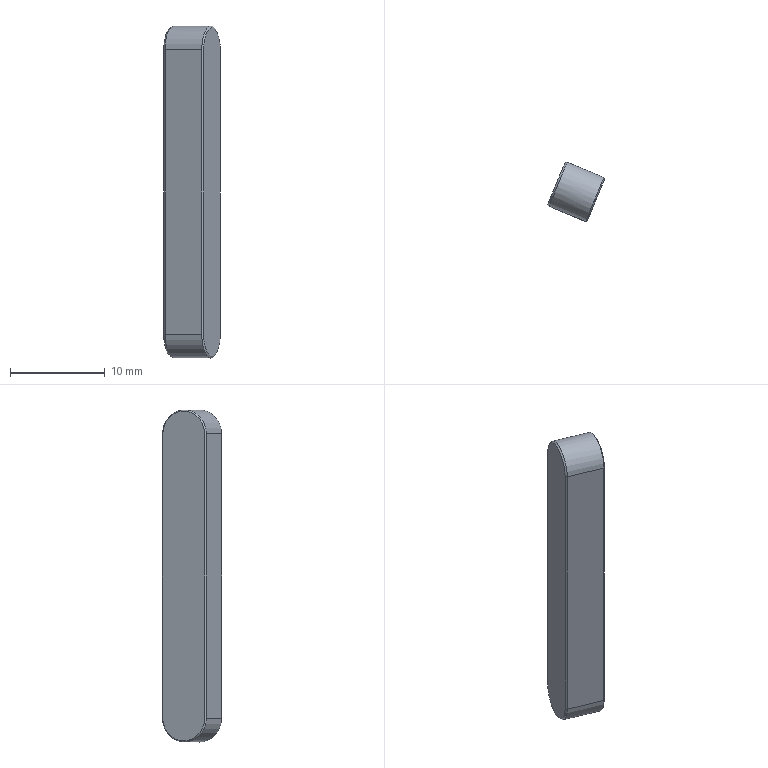Component | SolidWorks | 170423A4-ConveyorSynchronousPulleyAssembly-1_170423A4-Key5x30-1 | 1 solid | 17 faces | box 5.95 x 6.22 x 35 mm | volume 762 mm3 | plane 8 | cone 6 | cylinder 3 | commonest cylinder face diameters 5 x3
build123d program:
from build123d import *
from OCP.BRepFilletAPI import BRepFilletAPI_MakeChamfer

# Parameters (mm, degrees)
BOSS_EXTRUDE1_DEPTH = 4.5
CHAMFER1_SIZE       = 0.2
CHAMFER1_SIZE2      = 0.1155


with BuildPart() as part:
    # Sketch1 → Boss-Extrude1 (new body)
    with BuildSketch(Plane.XY):
        with BuildLine():
            Line((-15, 2.5), (15, 2.5))
            ThreePointArc((15, 2.5), (17.5, 0), (15, -2.5))
            Line((15, -2.5), (-15, -2.5))
            ThreePointArc((-15, -2.5), (-17.5, 0), (-15, 2.5))
        make_face()
    extrude(amount=BOSS_EXTRUDE1_DEPTH)

    # Chamfer1: one chamfer whose edges measure the first distance from different faces: ONE call of the kernel's chamfer builder (chamfer() names one face for all edges)
    chamfer1_edges_1 = [part.edges().sort_by_distance(p)[0] for p in [
        (17.5, 0, 4.5),
    ]]
    chamfer1_side_1 = [part.faces().sort_by_distance(p)[0] for p in [
        (17.5, 0, 2.25),
    ]]
    chamfer1_edges_2 = [part.edges().sort_by_distance(p)[0] for p in [
        (0, 2.5, 4.5),
    ]]
    chamfer1_side_2 = [part.faces().sort_by_distance(p)[0] for p in [
        (0, 2.5, 2.25),
    ]]
    chamfer1_edges_3 = [part.edges().sort_by_distance(p)[0] for p in [
        (-17.5, 0, 4.5),
    ]]
    chamfer1_side_3 = [part.faces().sort_by_distance(p)[0] for p in [
        (-17.5, 0, 2.25),
    ]]
    chamfer1_edges_4 = [part.edges().sort_by_distance(p)[0] for p in [
        (0, 2.5, 0),
        (17.5, 0, 0),
        (0, -2.5, 0),
        (-17.5, 0, 0),
    ]]
    chamfer1_side_4 = [part.faces().sort_by_distance(p)[0] for p in [
        (0, 0, 0),
    ]]
    chamfer1_edges_5 = [part.edges().sort_by_distance(p)[0] for p in [
        (0, -2.5, 4.5),
    ]]
    chamfer1_side_5 = [part.faces().sort_by_distance(p)[0] for p in [
        (0, -2.5, 2.25),
    ]]
    chamfer1 = BRepFilletAPI_MakeChamfer(part.part.solid().wrapped)
    for e in chamfer1_edges_1:
        chamfer1.Add(CHAMFER1_SIZE, CHAMFER1_SIZE2, e.wrapped, chamfer1_side_1[0].wrapped)  # the first distance lies on this face
    for e in chamfer1_edges_2:
        chamfer1.Add(CHAMFER1_SIZE, CHAMFER1_SIZE2, e.wrapped, chamfer1_side_2[0].wrapped)  # the first distance lies on this face
    for e in chamfer1_edges_3:
        chamfer1.Add(CHAMFER1_SIZE, CHAMFER1_SIZE2, e.wrapped, chamfer1_side_3[0].wrapped)  # the first distance lies on this face
    for e in chamfer1_edges_4:
        chamfer1.Add(CHAMFER1_SIZE, CHAMFER1_SIZE2, e.wrapped, chamfer1_side_4[0].wrapped)  # the first distance lies on this face
    for e in chamfer1_edges_5:
        chamfer1.Add(CHAMFER1_SIZE, CHAMFER1_SIZE2, e.wrapped, chamfer1_side_5[0].wrapped)  # the first distance lies on this face
    add(Compound.cast(chamfer1.Shape()), mode=Mode.REPLACE)


solid = part.part

# Placed as in the assembly
solid = solid.moved(Location((108.067, -124.236, 444), (-90, -67.477, -90)))
STEP:
#1=COLOUR_RGB('',0.7922,0.8196,0.9333);
#2=FILL_AREA_STYLE_COLOUR('',#1);
#3=FILL_AREA_STYLE('',(#2));
#4=SURFACE_STYLE_FILL_AREA(#3);
#5=SURFACE_SIDE_STYLE('',(#4));
#6=SURFACE_STYLE_USAGE(.BOTH.,#5);
#7=PRESENTATION_STYLE_ASSIGNMENT((#6));
#8=CARTESIAN_POINT('',(4.091,-4.823,16.796));
#9=VERTEX_POINT('',#8);
#10=CARTESIAN_POINT('',(4.055,-4.91,16.89));
#11=VERTEX_POINT('',#10);
#12=CARTESIAN_POINT('',(4.091,-4.823,16.89));
#13=DIRECTION('',(-0.9237,0.383,0.));
#14=DIRECTION('',(0.,-0.,1.));
#15=AXIS2_PLACEMENT_3D('',#12,#13,#14);
#16=CIRCLE('',#15,0.09388);
#17=EDGE_CURVE('',#9,#11,#16,.T.);
#18=ORIENTED_EDGE('',*,*,#17,.F.);
#19=CARTESIAN_POINT('',(4.098,-4.826,16.791));
#20=VERTEX_POINT('',#19);
#21=CARTESIAN_POINT('',(4.091,-4.823,16.796));
#22=DIRECTION('',(0.8,-0.3317,-0.5));
#23=VECTOR('',#22,39.37);
#24=LINE('',#21,#23);
#25=EDGE_CURVE('',#9,#20,#24,.T.);
#26=ORIENTED_EDGE('',*,*,#25,.T.);
#27=CARTESIAN_POINT('',(4.061,-4.917,16.89));
#28=VERTEX_POINT('',#27);
#29=CARTESIAN_POINT('',(4.098,-4.826,16.89));
#30=DIRECTION('',(0.9237,-0.383,-0.));
#31=DIRECTION('',(0.,-0.,1.));
#32=AXIS2_PLACEMENT_3D('',#29,#30,#31);
#33=CIRCLE('',#32,0.09843);
#34=EDGE_CURVE('',#28,#20,#33,.T.);
#35=ORIENTED_EDGE('',*,*,#34,.F.);
#36=CARTESIAN_POINT('',(4.061,-4.917,16.89));
#37=DIRECTION('',(-0.6084,0.7936,0.));
#38=VECTOR('',#37,39.37);
#39=LINE('',#36,#38);
#40=EDGE_CURVE('',#28,#11,#39,.T.);
#41=ORIENTED_EDGE('',*,*,#40,.T.);
#42=EDGE_LOOP('',(#18,#26,#35,#41));
#43=FACE_OUTER_BOUND('',#42,.T.);
#44=CARTESIAN_POINT('',(4.091,-4.823,16.89));
#45=DIRECTION('',(0.9237,-0.383,-0.));
#46=DIRECTION('',(0.,0.,-1.));
#47=AXIS2_PLACEMENT_3D('',#44,#45,#46);
#48=CONICAL_SURFACE('',#47,0.09388,0.5236);
#49=ADVANCED_FACE('',(#43),#48,.T.);
#50=CARTESIAN_POINT('',(4.255,-4.891,18.161));
#51=VERTEX_POINT('',#50);
#52=CARTESIAN_POINT('',(4.22,-4.975,18.071));
#53=VERTEX_POINT('',#52);
#54=CARTESIAN_POINT('',(4.255,-4.891,18.071));
#55=DIRECTION('',(0.9237,-0.383,-0.));
#56=DIRECTION('',(0.,-0.,1.));
#57=AXIS2_PLACEMENT_3D('',#54,#55,#56);
#58=CIRCLE('',#57,0.09055);
#59=EDGE_CURVE('',#51,#53,#58,.T.);
#60=ORIENTED_EDGE('',*,*,#59,.F.);
#61=CARTESIAN_POINT('',(4.25,-4.889,18.169));
#62=VERTEX_POINT('',#61);
#63=CARTESIAN_POINT('',(4.25,-4.889,18.169));
#64=DIRECTION('',(-0.4619,0.1915,0.866));
#65=VECTOR('',#64,39.37);
#66=LINE('',#63,#65);
#67=EDGE_CURVE('',#51,#62,#66,.T.);
#68=ORIENTED_EDGE('',*,*,#67,.T.);
#69=CARTESIAN_POINT('',(4.213,-4.98,18.071));
#70=VERTEX_POINT('',#69);
#71=CARTESIAN_POINT('',(4.25,-4.889,18.071));
#72=DIRECTION('',(-0.9237,0.383,0.));
#73=DIRECTION('',(0.,-0.,1.));
#74=AXIS2_PLACEMENT_3D('',#71,#72,#73);
#75=CIRCLE('',#74,0.09843);
#76=EDGE_CURVE('',#70,#62,#75,.T.);
#77=ORIENTED_EDGE('',*,*,#76,.F.);
#78=CARTESIAN_POINT('',(4.22,-4.975,18.071));
#79=DIRECTION('',(-0.7936,-0.6084,-0.));
#80=VECTOR('',#79,39.37);
#81=LINE('',#78,#80);
#82=EDGE_CURVE('',#53,#70,#81,.T.);
#83=ORIENTED_EDGE('',*,*,#82,.F.);
#84=EDGE_LOOP('',(#60,#68,#77,#83));
#85=FACE_OUTER_BOUND('',#84,.T.);
#86=CARTESIAN_POINT('',(4.25,-4.889,18.071));
#87=DIRECTION('',(-0.9237,0.383,0.));
#88=DIRECTION('',(0.,-0.,1.));
#89=AXIS2_PLACEMENT_3D('',#86,#87,#88);
#90=CONICAL_SURFACE('',#89,0.09843,1.047);
#91=ADVANCED_FACE('',(#85),#90,.T.);
#92=ORIENTED_EDGE('',*,*,#34,.T.);
#93=CARTESIAN_POINT('',(4.25,-4.889,16.791));
#94=VERTEX_POINT('',#93);
#95=CARTESIAN_POINT('',(4.091,-4.823,16.791));
#96=DIRECTION('',(0.9237,-0.383,-0.));
#97=VECTOR('',#96,39.37);
#98=LINE('',#95,#97);
#99=EDGE_CURVE('',#20,#94,#98,.T.);
#100=ORIENTED_EDGE('',*,*,#99,.T.);
#101=CARTESIAN_POINT('',(4.213,-4.98,16.89));
#102=VERTEX_POINT('',#101);
#103=CARTESIAN_POINT('',(4.25,-4.889,16.89));
#104=DIRECTION('',(-0.9237,0.383,0.));
#105=DIRECTION('',(0.,-0.,1.));
#106=AXIS2_PLACEMENT_3D('',#103,#104,#105);
#107=CIRCLE('',#106,0.09843);
#108=EDGE_CURVE('',#94,#102,#107,.T.);
#109=ORIENTED_EDGE('',*,*,#108,.T.);
#110=CARTESIAN_POINT('',(4.053,-4.914,16.89));
#111=DIRECTION('',(0.9237,-0.383,-0.));
#112=VECTOR('',#111,39.37);
#113=LINE('',#110,#112);
#114=EDGE_CURVE('',#28,#102,#113,.T.);
#115=ORIENTED_EDGE('',*,*,#114,.F.);
#116=EDGE_LOOP('',(#92,#100,#109,#115));
#117=FACE_OUTER_BOUND('',#116,.T.);
#118=CARTESIAN_POINT('',(4.091,-4.823,16.89));
#119=DIRECTION('',(0.9237,-0.383,-0.));
#120=DIRECTION('',(0.,0.,-1.));
#121=AXIS2_PLACEMENT_3D('',#118,#119,#120);
#122=CYLINDRICAL_SURFACE('',#121,0.09843);
#123=ADVANCED_FACE('',(#117),#122,.T.);
#124=ORIENTED_EDGE('',*,*,#99,.F.);
#125=CARTESIAN_POINT('',(4.136,-4.735,16.89));
#126=VERTEX_POINT('',#125);
#127=CARTESIAN_POINT('',(4.098,-4.826,16.89));
#128=DIRECTION('',(0.9237,-0.383,-0.));
#129=DIRECTION('',(0.,-0.,1.));
#130=AXIS2_PLACEMENT_3D('',#127,#128,#129);
#131=CIRCLE('',#130,0.09843);
#132=EDGE_CURVE('',#20,#126,#131,.T.);
#133=ORIENTED_EDGE('',*,*,#132,.T.);
#134=CARTESIAN_POINT('',(4.288,-4.799,16.89));
#135=VERTEX_POINT('',#134);
#136=CARTESIAN_POINT('',(4.129,-4.732,16.89));
#137=DIRECTION('',(0.9237,-0.383,-0.));
#138=VECTOR('',#137,39.37);
#139=LINE('',#136,#138);
#140=EDGE_CURVE('',#126,#135,#139,.T.);
#141=ORIENTED_EDGE('',*,*,#140,.T.);
#142=CARTESIAN_POINT('',(4.25,-4.889,16.89));
#143=DIRECTION('',(-0.9237,0.383,0.));
#144=DIRECTION('',(0.,-0.,1.));
#145=AXIS2_PLACEMENT_3D('',#142,#143,#144);
#146=CIRCLE('',#145,0.09843);
#147=EDGE_CURVE('',#135,#94,#146,.T.);
#148=ORIENTED_EDGE('',*,*,#147,.T.);
#149=EDGE_LOOP('',(#124,#133,#141,#148));
#150=FACE_OUTER_BOUND('',#149,.T.);
#151=CARTESIAN_POINT('',(4.091,-4.823,16.89));
#152=DIRECTION('',(0.9237,-0.383,-0.));
#153=DIRECTION('',(0.,0.,-1.));
#154=AXIS2_PLACEMENT_3D('',#151,#152,#153);
#155=CYLINDRICAL_SURFACE('',#154,0.09843);
#156=ADVANCED_FACE('',(#150),#155,.T.);
#157=ORIENTED_EDGE('',*,*,#114,.T.);
#158=CARTESIAN_POINT('',(4.213,-4.98,16.89));
#159=DIRECTION('',(0.,-0.,1.));
#160=VECTOR('',#159,39.37);
#161=LINE('',#158,#160);
#162=EDGE_CURVE('',#102,#70,#161,.T.);
#163=ORIENTED_EDGE('',*,*,#162,.T.);
#164=CARTESIAN_POINT('',(4.061,-4.917,18.071));
#165=VERTEX_POINT('',#164);
#166=CARTESIAN_POINT('',(4.053,-4.914,18.071));
#167=DIRECTION('',(0.9237,-0.383,-0.));
#168=VECTOR('',#167,39.37);
#169=LINE('',#166,#168);
#170=EDGE_CURVE('',#165,#70,#169,.T.);
#171=ORIENTED_EDGE('',*,*,#170,.F.);
#172=CARTESIAN_POINT('',(4.061,-4.917,16.89));
#173=DIRECTION('',(-0.,0.,-1.));
#174=VECTOR('',#173,39.37);
#175=LINE('',#172,#174);
#176=EDGE_CURVE('',#165,#28,#175,.T.);
#177=ORIENTED_EDGE('',*,*,#176,.T.);
#178=EDGE_LOOP('',(#157,#163,#171,#177));
#179=FACE_OUTER_BOUND('',#178,.T.);
#180=CARTESIAN_POINT('',(4.053,-4.914,16.89));
#181=DIRECTION('',(0.383,0.9237,0.));
#182=DIRECTION('',(-0.9237,0.383,0.));
#183=AXIS2_PLACEMENT_3D('',#180,#181,#182);
#184=PLANE('',#183);
#185=ADVANCED_FACE('',(#179),#184,.F.);
#186=ORIENTED_EDGE('',*,*,#170,.T.);
#187=ORIENTED_EDGE('',*,*,#76,.T.);
#188=CARTESIAN_POINT('',(4.288,-4.799,18.071));
#189=VERTEX_POINT('',#188);
#190=CARTESIAN_POINT('',(4.25,-4.889,18.071));
#191=DIRECTION('',(-0.9237,0.383,0.));
#192=DIRECTION('',(0.,-0.,1.));
#193=AXIS2_PLACEMENT_3D('',#190,#191,#192);
#194=CIRCLE('',#193,0.09843);
#195=EDGE_CURVE('',#62,#189,#194,.T.);
#196=ORIENTED_EDGE('',*,*,#195,.T.);
#197=CARTESIAN_POINT('',(4.136,-4.735,18.071));
#198=VERTEX_POINT('',#197);
#199=CARTESIAN_POINT('',(4.129,-4.732,18.071));
#200=DIRECTION('',(0.9237,-0.383,-0.));
#201=VECTOR('',#200,39.37);
#202=LINE('',#199,#201);
#203=EDGE_CURVE('',#198,#189,#202,.T.);
#204=ORIENTED_EDGE('',*,*,#203,.F.);
#205=CARTESIAN_POINT('',(4.098,-4.826,18.071));
#206=DIRECTION('',(0.9237,-0.383,-0.));
#207=DIRECTION('',(0.,-0.,1.));
#208=AXIS2_PLACEMENT_3D('',#205,#206,#207);
#209=CIRCLE('',#208,0.09843);
#210=EDGE_CURVE('',#198,#165,#209,.T.);
#211=ORIENTED_EDGE('',*,*,#210,.T.);
#212=EDGE_LOOP('',(#186,#187,#196,#204,#211));
#213=FACE_OUTER_BOUND('',#212,.T.);
#214=CARTESIAN_POINT('',(4.091,-4.823,18.071));
#215=DIRECTION('',(0.9237,-0.383,-0.));
#216=DIRECTION('',(0.,0.,-1.));
#217=AXIS2_PLACEMENT_3D('',#214,#215,#216);
#218=CYLINDRICAL_SURFACE('',#217,0.09843);
#219=ADVANCED_FACE('',(#213),#218,.T.);
#220=ORIENTED_EDGE('',*,*,#203,.T.);
#221=CARTESIAN_POINT('',(4.288,-4.799,16.89));
#222=DIRECTION('',(-0.,0.,-1.));
#223=VECTOR('',#222,39.37);
#224=LINE('',#221,#223);
#225=EDGE_CURVE('',#189,#135,#224,.T.);
#226=ORIENTED_EDGE('',*,*,#225,.T.);
#227=ORIENTED_EDGE('',*,*,#140,.F.);
#228=CARTESIAN_POINT('',(4.136,-4.735,18.071));
#229=DIRECTION('',(0.,-0.,1.));
#230=VECTOR('',#229,39.37);
#231=LINE('',#228,#230);
#232=EDGE_CURVE('',#126,#198,#231,.T.);
#233=ORIENTED_EDGE('',*,*,#232,.T.);
#234=EDGE_LOOP('',(#220,#226,#227,#233));
#235=FACE_OUTER_BOUND('',#234,.T.);
#236=CARTESIAN_POINT('',(4.129,-4.732,16.89));
#237=DIRECTION('',(-0.383,-0.9237,-0.));
#238=DIRECTION('',(0.,-0.,1.));
#239=AXIS2_PLACEMENT_3D('',#236,#237,#238);
#240=PLANE('',#239);
#241=ADVANCED_FACE('',(#235),#240,.F.);
#242=CARTESIAN_POINT('',(4.055,-4.91,18.071));
#243=VERTEX_POINT('',#242);
#244=CARTESIAN_POINT('',(4.127,-4.737,18.071));
#245=VERTEX_POINT('',#244);
#246=CARTESIAN_POINT('',(4.091,-4.823,18.071));
#247=DIRECTION('',(-0.9237,0.383,0.));
#248=DIRECTION('',(0.,-0.,1.));
#249=AXIS2_PLACEMENT_3D('',#246,#247,#248);
#250=CIRCLE('',#249,0.09388);
#251=EDGE_CURVE('',#243,#245,#250,.T.);
#252=ORIENTED_EDGE('',*,*,#251,.T.);
#253=CARTESIAN_POINT('',(4.127,-4.737,16.89));
#254=VERTEX_POINT('',#253);
#255=CARTESIAN_POINT('',(4.127,-4.737,16.89));
#256=DIRECTION('',(-0.,0.,-1.));
#257=VECTOR('',#256,39.37);
#258=LINE('',#255,#257);
#259=EDGE_CURVE('',#245,#254,#258,.T.);
#260=ORIENTED_EDGE('',*,*,#259,.T.);
#261=CARTESIAN_POINT('',(4.091,-4.823,16.89));
#262=DIRECTION('',(-0.9237,0.383,0.));
#263=DIRECTION('',(0.,-0.,1.));
#264=AXIS2_PLACEMENT_3D('',#261,#262,#263);
#265=CIRCLE('',#264,0.09388);
#266=EDGE_CURVE('',#254,#9,#265,.T.);
#267=ORIENTED_EDGE('',*,*,#266,.T.);
#268=ORIENTED_EDGE('',*,*,#17,.T.);
#269=CARTESIAN_POINT('',(4.055,-4.91,18.071));
#270=DIRECTION('',(0.,-0.,1.));
#271=VECTOR('',#270,39.37);
#272=LINE('',#269,#271);
#273=EDGE_CURVE('',#11,#243,#272,.T.);
#274=ORIENTED_EDGE('',*,*,#273,.T.);
#275=EDGE_LOOP('',(#252,#260,#267,#268,#274));
#276=FACE_OUTER_BOUND('',#275,.T.);
#277=CARTESIAN_POINT('',(4.091,-4.823,16.89));
#278=DIRECTION('',(-0.9237,0.383,0.));
#279=DIRECTION('',(0.,-0.,1.));
#280=AXIS2_PLACEMENT_3D('',#277,#278,#279);
#281=PLANE('',#280);
#282=ADVANCED_FACE('',(#276),#281,.T.);
#283=CARTESIAN_POINT('',(4.289,-4.808,18.071));
#284=VERTEX_POINT('',#283);
#285=CARTESIAN_POINT('',(4.255,-4.891,18.071));
#286=DIRECTION('',(0.9237,-0.383,-0.));
#287=DIRECTION('',(0.,-0.,1.));
#288=AXIS2_PLACEMENT_3D('',#285,#286,#287);
#289=CIRCLE('',#288,0.09055);
#290=EDGE_CURVE('',#284,#51,#289,.T.);
#291=ORIENTED_EDGE('',*,*,#290,.T.);
#292=ORIENTED_EDGE('',*,*,#59,.T.);
#293=CARTESIAN_POINT('',(4.22,-4.975,16.89));
#294=VERTEX_POINT('',#293);
#295=CARTESIAN_POINT('',(4.22,-4.975,16.89));
#296=DIRECTION('',(-0.,0.,-1.));
#297=VECTOR('',#296,39.37);
#298=LINE('',#295,#297);
#299=EDGE_CURVE('',#53,#294,#298,.T.);
#300=ORIENTED_EDGE('',*,*,#299,.T.);
#301=CARTESIAN_POINT('',(4.289,-4.808,16.89));
#302=VERTEX_POINT('',#301);
#303=CARTESIAN_POINT('',(4.255,-4.891,16.89));
#304=DIRECTION('',(0.9237,-0.383,-0.));
#305=DIRECTION('',(0.,-0.,1.));
#306=AXIS2_PLACEMENT_3D('',#303,#304,#305);
#307=CIRCLE('',#306,0.09055);
#308=EDGE_CURVE('',#294,#302,#307,.T.);
#309=ORIENTED_EDGE('',*,*,#308,.T.);
#310=CARTESIAN_POINT('',(4.289,-4.808,16.89));
#311=DIRECTION('',(0.,-0.,1.));
#312=VECTOR('',#311,39.37);
#313=LINE('',#310,#312);
#314=EDGE_CURVE('',#302,#284,#313,.T.);
#315=ORIENTED_EDGE('',*,*,#314,.T.);
#316=EDGE_LOOP('',(#291,#292,#300,#309,#315));
#317=FACE_OUTER_BOUND('',#316,.T.);
#318=CARTESIAN_POINT('',(4.255,-4.891,16.89));
#319=DIRECTION('',(-0.9237,0.383,0.));
#320=DIRECTION('',(0.,-0.,1.));
#321=AXIS2_PLACEMENT_3D('',#318,#319,#320);
#322=PLANE('',#321);
#323=ADVANCED_FACE('',(#317),#322,.F.);
#324=CARTESIAN_POINT('',(4.289,-4.808,18.071));
#325=DIRECTION('',(-0.1301,0.9915,0.));
#326=VECTOR('',#325,39.37);
#327=LINE('',#324,#326);
#328=EDGE_CURVE('',#284,#189,#327,.T.);
#329=ORIENTED_EDGE('',*,*,#328,.F.);
#330=ORIENTED_EDGE('',*,*,#314,.F.);
#331=CARTESIAN_POINT('',(4.288,-4.799,16.89));
#332=DIRECTION('',(0.1301,-0.9915,-0.));
#333=VECTOR('',#332,39.37);
#334=LINE('',#331,#333);
#335=EDGE_CURVE('',#135,#302,#334,.T.);
#336=ORIENTED_EDGE('',*,*,#335,.F.);
#337=ORIENTED_EDGE('',*,*,#225,.F.);
#338=EDGE_LOOP('',(#329,#330,#336,#337));
#339=FACE_OUTER_BOUND('',#338,.T.);
#340=CARTESIAN_POINT('',(4.288,-4.799,16.89));
#341=DIRECTION('',(-0.9915,-0.1301,-0.));
#342=DIRECTION('',(-0.,0.,-1.));
#343=AXIS2_PLACEMENT_3D('',#340,#341,#342);
#344=PLANE('',#343);
#345=ADVANCED_FACE('',(#339),#344,.F.);
#346=ORIENTED_EDGE('',*,*,#335,.T.);
#347=ORIENTED_EDGE('',*,*,#308,.F.);
#348=CARTESIAN_POINT('',(4.213,-4.98,16.89));
#349=DIRECTION('',(0.7936,0.6084,0.));
#350=VECTOR('',#349,39.37);
#351=LINE('',#348,#350);
#352=EDGE_CURVE('',#102,#294,#351,.T.);
#353=ORIENTED_EDGE('',*,*,#352,.F.);
#354=ORIENTED_EDGE('',*,*,#108,.F.);
#355=ORIENTED_EDGE('',*,*,#147,.F.);
#356=EDGE_LOOP('',(#346,#347,#353,#354,#355));
#357=FACE_OUTER_BOUND('',#356,.T.);
#358=CARTESIAN_POINT('',(4.25,-4.889,16.89));
#359=DIRECTION('',(-0.9237,0.383,0.));
#360=DIRECTION('',(0.,-0.,1.));
#361=AXIS2_PLACEMENT_3D('',#358,#359,#360);
#362=CONICAL_SURFACE('',#361,0.09843,1.047);
#363=ADVANCED_FACE('',(#357),#362,.T.);
#364=ORIENTED_EDGE('',*,*,#67,.F.);
#365=ORIENTED_EDGE('',*,*,#290,.F.);
#366=ORIENTED_EDGE('',*,*,#328,.T.);
#367=ORIENTED_EDGE('',*,*,#195,.F.);
#368=EDGE_LOOP('',(#364,#365,#366,#367));
#369=FACE_OUTER_BOUND('',#368,.T.);
#370=CARTESIAN_POINT('',(4.25,-4.889,18.071));
#371=DIRECTION('',(-0.9237,0.383,0.));
#372=DIRECTION('',(0.,-0.,1.));
#373=AXIS2_PLACEMENT_3D('',#370,#371,#372);
#374=CONICAL_SURFACE('',#373,0.09843,1.047);
#375=ADVANCED_FACE('',(#369),#374,.T.);
#376=ORIENTED_EDGE('',*,*,#352,.T.);
#377=ORIENTED_EDGE('',*,*,#299,.F.);
#378=ORIENTED_EDGE('',*,*,#82,.T.);
#379=ORIENTED_EDGE('',*,*,#162,.F.);
#380=EDGE_LOOP('',(#376,#377,#378,#379));
#381=FACE_OUTER_BOUND('',#380,.T.);
#382=CARTESIAN_POINT('',(4.213,-4.98,16.89));
#383=DIRECTION('',(-0.6084,0.7936,0.));
#384=DIRECTION('',(0.,-0.,1.));
#385=AXIS2_PLACEMENT_3D('',#382,#383,#384);
#386=PLANE('',#385);
#387=ADVANCED_FACE('',(#381),#386,.F.);
#388=ORIENTED_EDGE('',*,*,#40,.F.);
#389=ORIENTED_EDGE('',*,*,#176,.F.);
#390=CARTESIAN_POINT('',(4.055,-4.91,18.071));
#391=DIRECTION('',(0.6084,-0.7936,-0.));
#392=VECTOR('',#391,39.37);
#393=LINE('',#390,#392);
#394=EDGE_CURVE('',#243,#165,#393,.T.);
#395=ORIENTED_EDGE('',*,*,#394,.F.);
#396=ORIENTED_EDGE('',*,*,#273,.F.);
#397=EDGE_LOOP('',(#388,#389,#395,#396));
#398=FACE_OUTER_BOUND('',#397,.T.);
#399=CARTESIAN_POINT('',(4.055,-4.91,16.89));
#400=DIRECTION('',(-0.7936,-0.6084,-0.));
#401=DIRECTION('',(-0.,0.,-1.));
#402=AXIS2_PLACEMENT_3D('',#399,#400,#401);
#403=PLANE('',#402);
#404=ADVANCED_FACE('',(#398),#403,.T.);
#405=ORIENTED_EDGE('',*,*,#394,.T.);
#406=ORIENTED_EDGE('',*,*,#210,.F.);
#407=CARTESIAN_POINT('',(4.127,-4.737,18.071));
#408=DIRECTION('',(0.9915,0.1301,0.));
#409=VECTOR('',#408,39.37);
#410=LINE('',#407,#409);
#411=EDGE_CURVE('',#245,#198,#410,.T.);
#412=ORIENTED_EDGE('',*,*,#411,.F.);
#413=ORIENTED_EDGE('',*,*,#251,.F.);
#414=EDGE_LOOP('',(#405,#406,#412,#413));
#415=FACE_OUTER_BOUND('',#414,.T.);
#416=CARTESIAN_POINT('',(4.091,-4.823,18.071));
#417=DIRECTION('',(0.9237,-0.383,-0.));
#418=DIRECTION('',(0.,0.,-1.));
#419=AXIS2_PLACEMENT_3D('',#416,#417,#418);
#420=CONICAL_SURFACE('',#419,0.09388,0.5236);
#421=ADVANCED_FACE('',(#415),#420,.T.);
#422=ORIENTED_EDGE('',*,*,#25,.F.);
#423=ORIENTED_EDGE('',*,*,#266,.F.);
#424=CARTESIAN_POINT('',(4.136,-4.735,16.89));
#425=DIRECTION('',(-0.9915,-0.1301,-0.));
#426=VECTOR('',#425,39.37);
#427=LINE('',#424,#426);
#428=EDGE_CURVE('',#126,#254,#427,.T.);
#429=ORIENTED_EDGE('',*,*,#428,.F.);
#430=ORIENTED_EDGE('',*,*,#132,.F.);
#431=EDGE_LOOP('',(#422,#423,#429,#430));
#432=FACE_OUTER_BOUND('',#431,.T.);
#433=CARTESIAN_POINT('',(4.091,-4.823,16.89));
#434=DIRECTION('',(0.9237,-0.383,-0.));
#435=DIRECTION('',(0.,0.,-1.));
#436=AXIS2_PLACEMENT_3D('',#433,#434,#435);
#437=CONICAL_SURFACE('',#436,0.09388,0.5236);
#438=ADVANCED_FACE('',(#432),#437,.T.);
#439=ORIENTED_EDGE('',*,*,#411,.T.);
#440=ORIENTED_EDGE('',*,*,#232,.F.);
#441=ORIENTED_EDGE('',*,*,#428,.T.);
#442=ORIENTED_EDGE('',*,*,#259,.F.);
#443=EDGE_LOOP('',(#439,#440,#441,#442));
#444=FACE_OUTER_BOUND('',#443,.T.);
#445=CARTESIAN_POINT('',(4.127,-4.737,16.89));
#446=DIRECTION('',(-0.1301,0.9915,0.));
#447=DIRECTION('',(0.,-0.,1.));
#448=AXIS2_PLACEMENT_3D('',#445,#446,#447);
#449=PLANE('',#448);
#450=ADVANCED_FACE('',(#444),#449,.T.);
#451=CLOSED_SHELL('',(#49,#91,#123,#156,#185,#219,#241,#282,#323,#345,#363,#375,#387,#404,#421,#438,#450));
#452=MANIFOLD_SOLID_BREP('',#451);
#453=STYLED_ITEM('',(#7),#452);
#454=(LENGTH_UNIT()NAMED_UNIT(*)SI_UNIT($,.METRE.));
#455=LENGTH_MEASURE_WITH_UNIT(LENGTH_MEASURE(0.0254),#454);
#456=DIMENSIONAL_EXPONENTS(1.,0.,0.,0.,0.,0.,0.);
#457=(CONVERSION_BASED_UNIT('',#455)LENGTH_UNIT()NAMED_UNIT(#456));
#458=UNCERTAINTY_MEASURE_WITH_UNIT(LENGTH_MEASURE(0.00001),#457,'','');
#459=(NAMED_UNIT(*)PLANE_ANGLE_UNIT()SI_UNIT($,.RADIAN.));
#460=(NAMED_UNIT(*)SI_UNIT($,.STERADIAN.)SOLID_ANGLE_UNIT());
#461=(GEOMETRIC_REPRESENTATION_CONTEXT(3)GLOBAL_UNCERTAINTY_ASSIGNED_CONTEXT((#458))GLOBAL_UNIT_ASSIGNED_CONTEXT((#457,#459,#460))REPRESENTATION_CONTEXT('',''));
#462=MECHANICAL_DESIGN_GEOMETRIC_PRESENTATION_REPRESENTATION('',(#453),#461);
#463=PRESENTATION_LAYER_ASSIGNMENT('','',(#453));
#464=CARTESIAN_POINT('',(0.,0.,0.));
#465=DIRECTION('',(0.,0.,1.));
#466=DIRECTION('',(1.,0.,0.));
#467=AXIS2_PLACEMENT_3D('',#464,#465,#466);
#468=(LENGTH_UNIT()NAMED_UNIT(*)SI_UNIT($,.METRE.));
#469=LENGTH_MEASURE_WITH_UNIT(LENGTH_MEASURE(0.0254),#468);
#470=DIMENSIONAL_EXPONENTS(1.,0.,0.,0.,0.,0.,0.);
#471=(CONVERSION_BASED_UNIT('',#469)LENGTH_UNIT()NAMED_UNIT(#470));
#472=UNCERTAINTY_MEASURE_WITH_UNIT(LENGTH_MEASURE(0.00001),#471,'','');
#473=(NAMED_UNIT(*)PLANE_ANGLE_UNIT()SI_UNIT($,.RADIAN.));
#474=(NAMED_UNIT(*)SI_UNIT($,.STERADIAN.)SOLID_ANGLE_UNIT());
#475=(GEOMETRIC_REPRESENTATION_CONTEXT(3)GLOBAL_UNCERTAINTY_ASSIGNED_CONTEXT((#472))GLOBAL_UNIT_ASSIGNED_CONTEXT((#471,#473,#474))REPRESENTATION_CONTEXT('',''));
#476=ADVANCED_BREP_SHAPE_REPRESENTATION('',(#452,#467),#475);